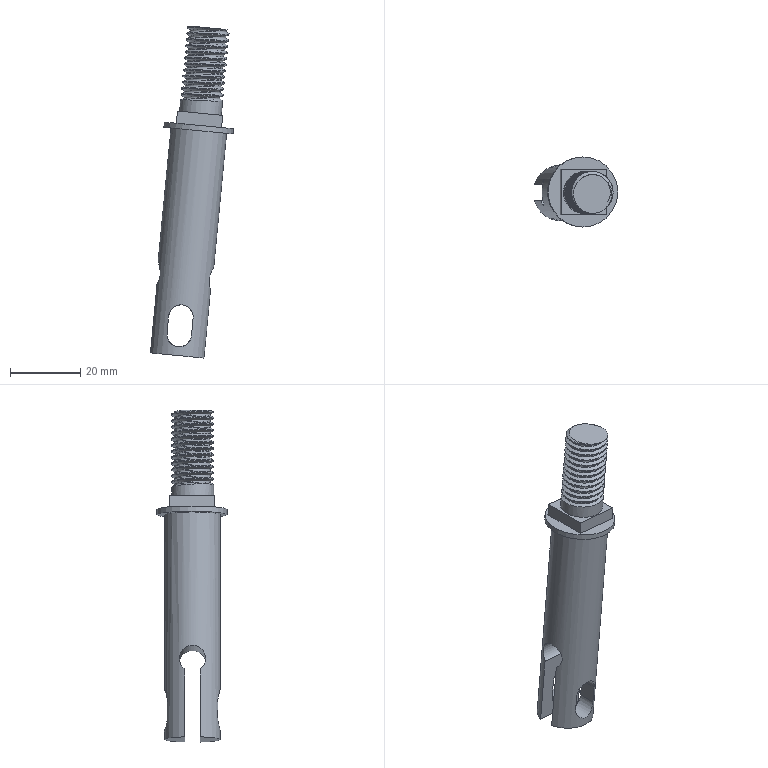Component | NX | DAOZHU | 1 solid | 39 faces | volume 13535 mm3 | cylinder 20 | plane 17 | spline 2 | commonest cylinder face diameters 12 x12 7 x4 16 x1 20 x1 7.5 x1 10.25 x1